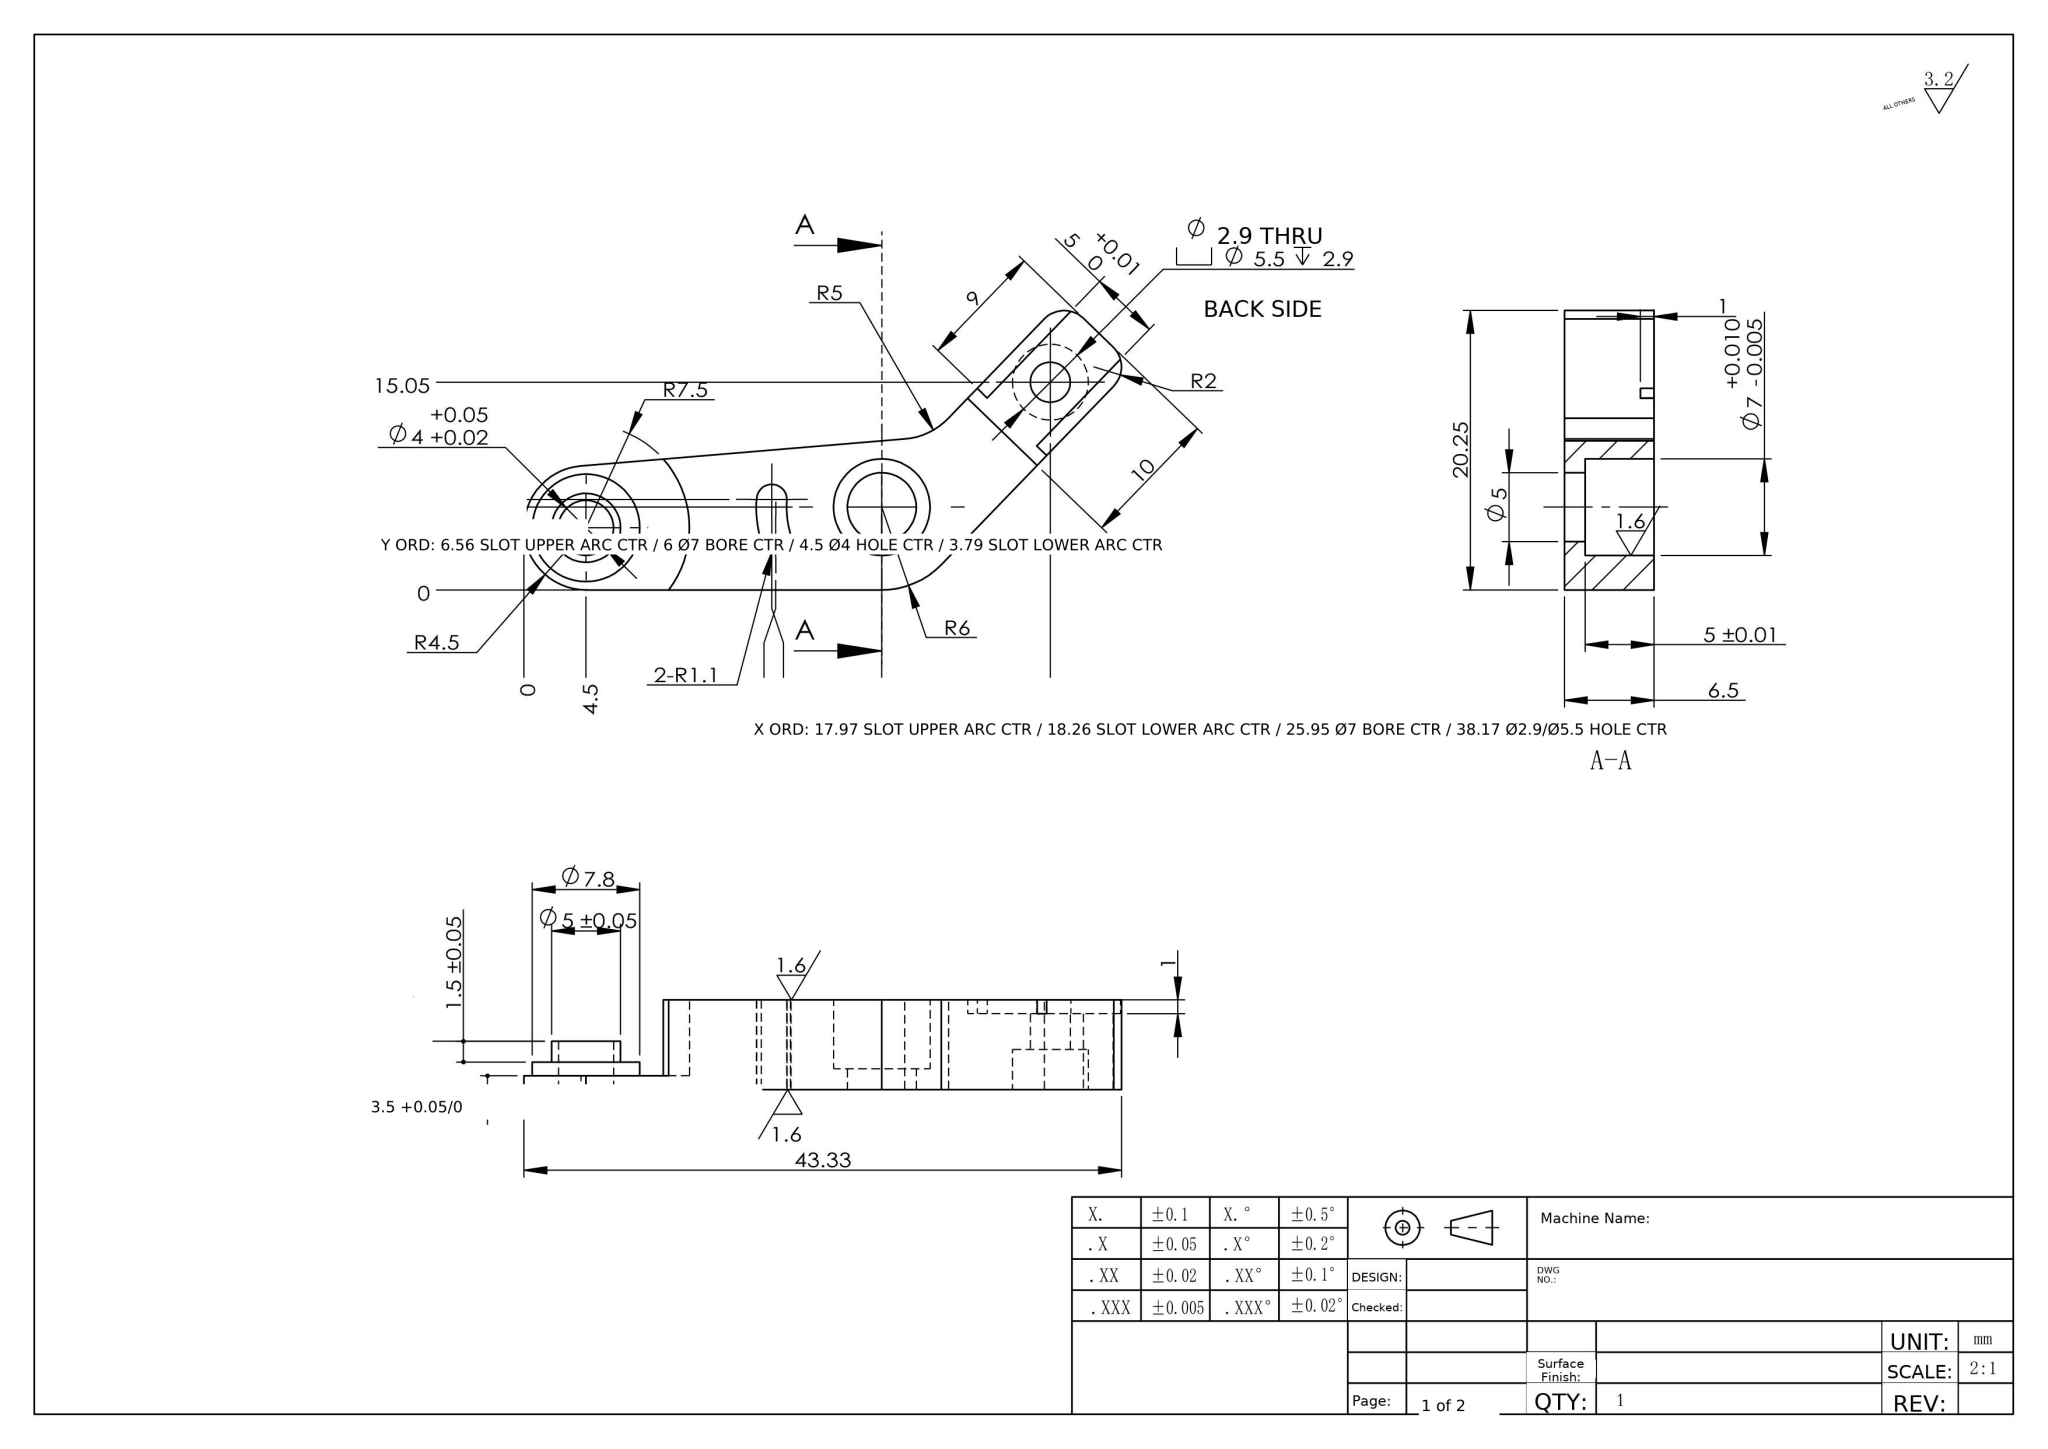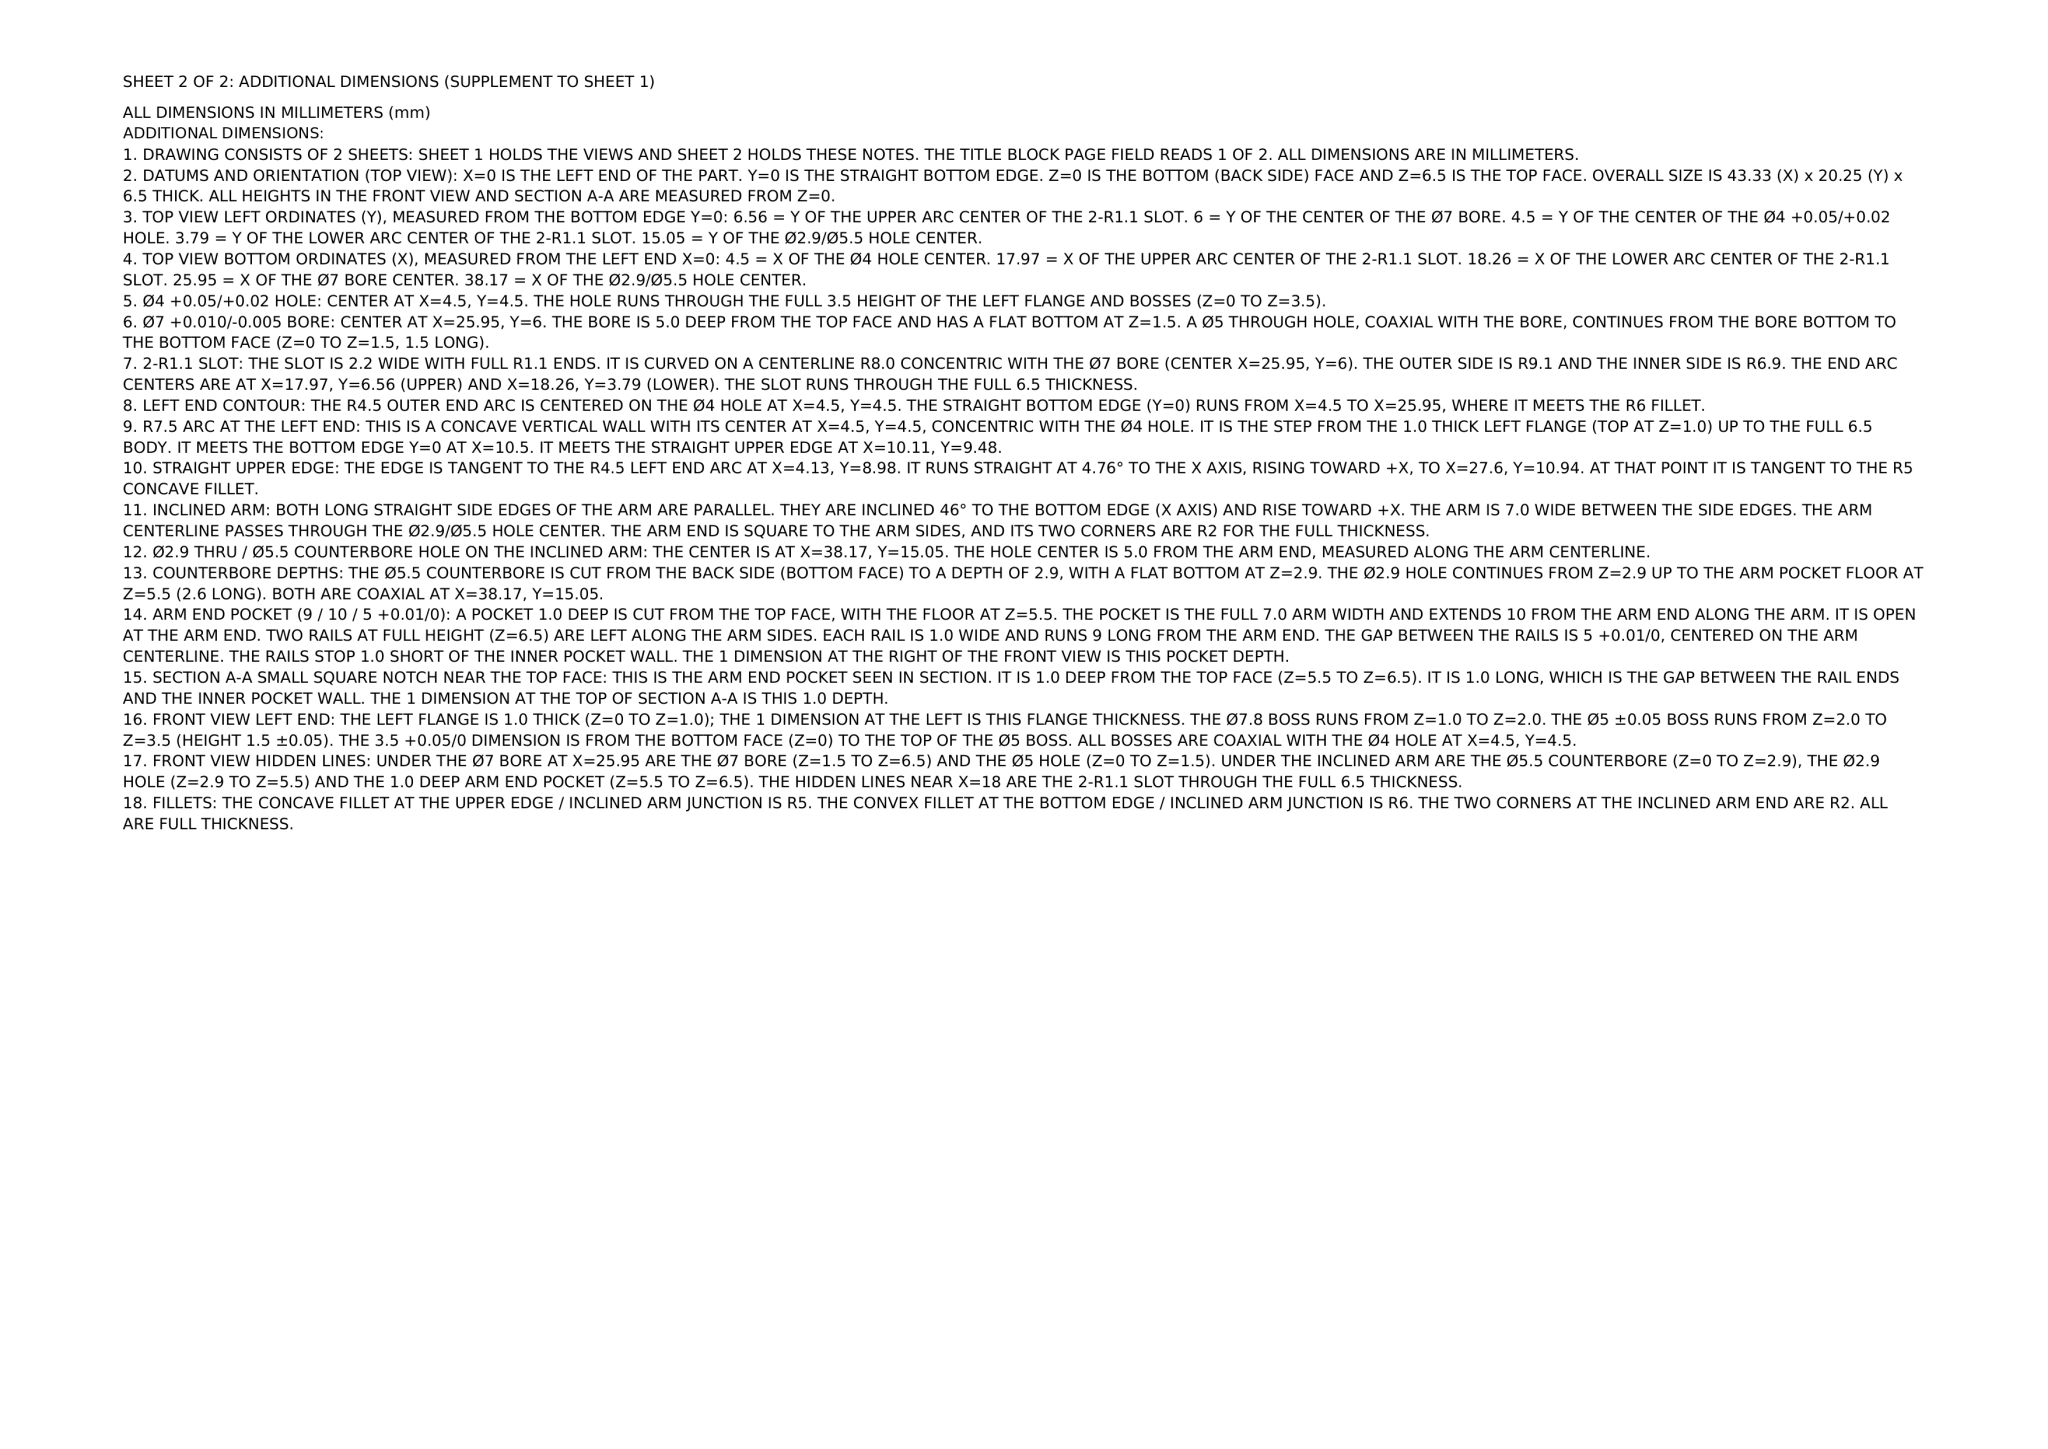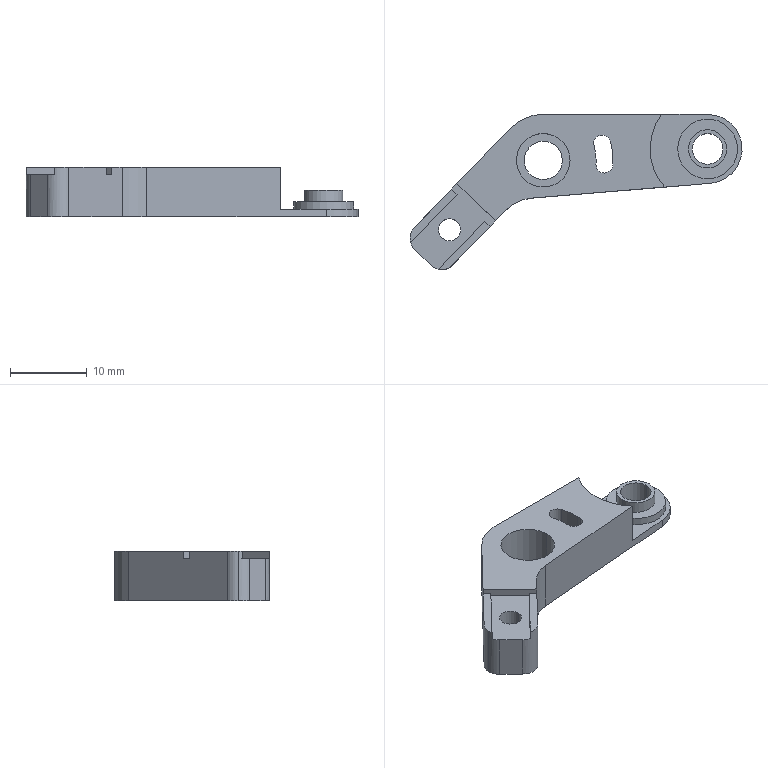Part | NX | mm | 1 solid | 48 faces | box 43.33 x 20.25 x 6.5 mm | volume 1697 mm3 | cylinder 28 | plane 20 | commonest cylinder face diameters 4 x5 5 x4 5.5 x2 2.9 x2 18.2 x2 13.8 x2 7 x2 15 x2